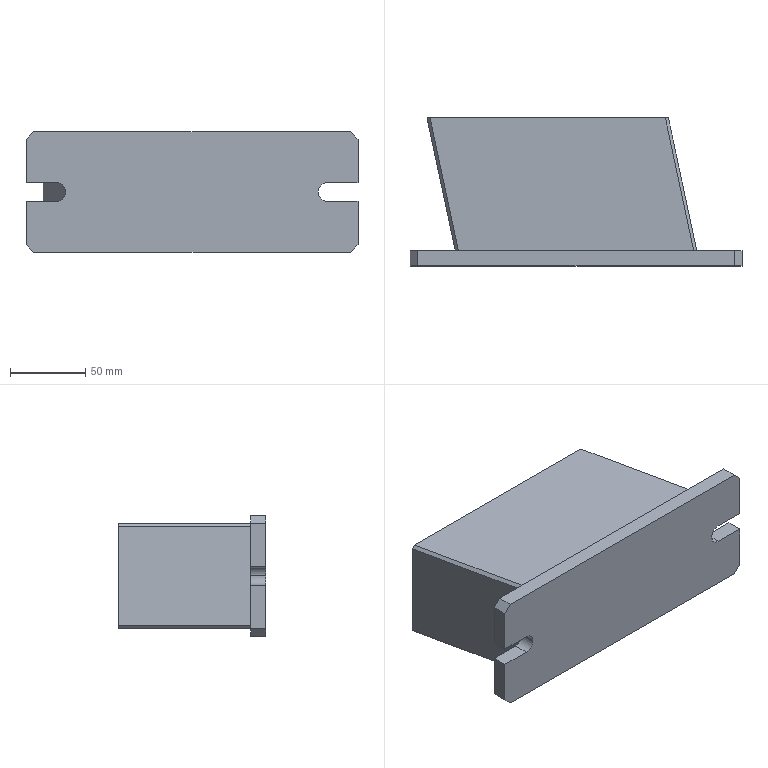Component | SolidWorks | 5160#x98x70StraightVibrator9.26-1 | 1 solid | 28 faces | box 220 x 98 x 80 mm | volume 1154153 mm3 | plane 25 | cylinder 3 | commonest cylinder face diameters 12.5 x3 | material AISI 1045 Steel, Cold Drawn
build123d program:
from build123d import *

# Parameters (mm, degrees)
BOSS_EXTRUDE1_DEPTH = 70
SKETCH2_W           = 220
SKETCH2_H           = 80
BOSS_EXTRUDE2_DEPTH = 10
CHAMFER1_SIZE       = 2
CUT_EXTRUDE1_DEPTH  = 207.666
CHAMFER2_SIZE       = 5


with BuildPart() as part:
    # Sketch1 → Boss-Extrude1 (new body)
    with BuildSketch(Plane.XY):
        Polygon((0, 0), (160, 0), (141.295, -88), (-18.705, -88), align=None)
    extrude(amount=BOSS_EXTRUDE1_DEPTH)

    # Sketch2 → Boss-Extrude2 (add)
    with BuildSketch(Plane.XZ.offset(88)):
        with Locations((61.295, 35)):
            Rectangle(SKETCH2_W, SKETCH2_H)
    extrude(amount=BOSS_EXTRUDE2_DEPTH)

    # Chamfer1
    chamfer1_edges = [part.edges().sort_by_distance(p)[0] for p in [
        (150.648, -44, 70),
        (-9.352, -44, 70),
        (150.648, -44, 0),
        (-9.352, -44, 0),
    ]]
    chamfer(chamfer1_edges, length=CHAMFER1_SIZE)

    # Sketch3 → Cut-Extrude1 (cut, through all)
    with BuildSketch(Plane(origin=(0, -88, 0), x_dir=(1, 0, 0), z_dir=(0, 1, 0))):
        with BuildLine():
            Line((-28.705, -41.25), (-48.705, -41.25))
            Line((-48.705, -41.25), (-48.705, -35))
            Line((-48.705, -35), (-48.705, -28.75))
            Line((-48.705, -28.75), (-28.705, -28.75))
            ThreePointArc((-28.705, -28.75), (-22.455, -35), (-28.705, -41.25))
        make_face()
        with BuildLine():
            Line((171.295, -28.75), (171.295, -35))
            Line((171.295, -35), (171.295, -41.25))
            Line((171.295, -41.25), (151.295, -41.25))
            ThreePointArc((151.295, -41.25), (145.045, -35), (151.295, -28.75))
            Line((151.295, -28.75), (171.295, -28.75))
        make_face()
    extrude(amount=-CUT_EXTRUDE1_DEPTH, mode=Mode.SUBTRACT)

    # Chamfer2
    chamfer2_edges = [part.edges().sort_by_distance(p)[0] for p in [
        (-48.705, -93, 75),
        (-48.705, -93, -5),
        (171.295, -93, -5),
        (171.295, -93, 75),
    ]]
    chamfer(chamfer2_edges, length=CHAMFER2_SIZE)


solid = part.part

# Placed as in the assembly
solid = solid.moved(Location((265, -185, 50.25), (-180, 0, 180)))